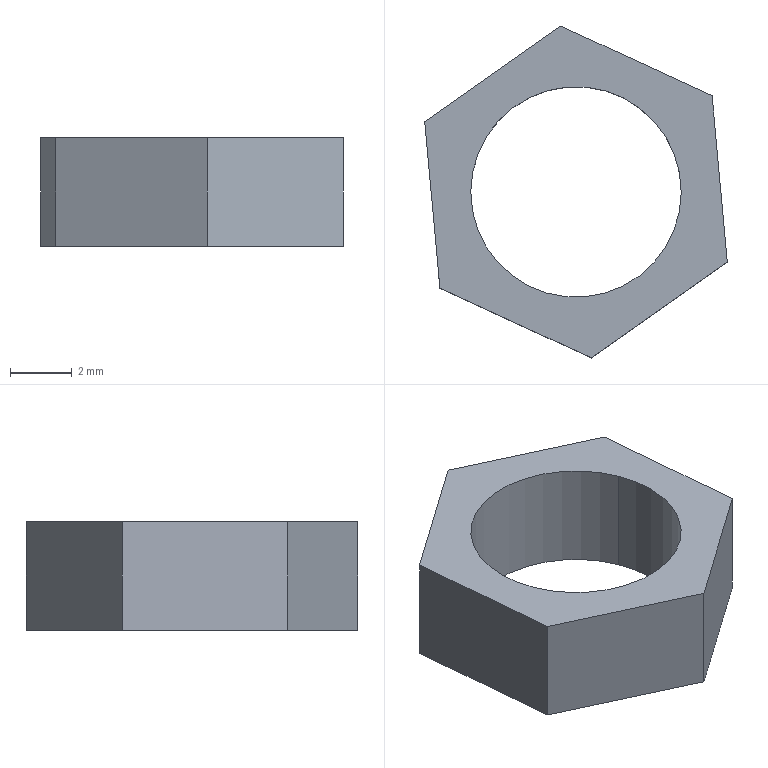Component | SolidWorks | ThinNut-1 | 1 solid | 10 faces | box 9.77 x 10.72 x 3.5 mm | volume 136 mm3 | plane 8 | cylinder 2 | commonest cylinder face diameters 6.8 x2
STEP:
#1=COLOUR_RGB('',0.7922,0.8196,0.9333);
#2=FILL_AREA_STYLE_COLOUR('',#1);
#3=FILL_AREA_STYLE('',(#2));
#4=SURFACE_STYLE_FILL_AREA(#3);
#5=SURFACE_SIDE_STYLE('',(#4));
#6=SURFACE_STYLE_USAGE(.BOTH.,#5);
#7=PRESENTATION_STYLE_ASSIGNMENT((#6));
#8=CARTESIAN_POINT('',(-4.037,-1.074,7.106));
#9=VERTEX_POINT('',#8);
#10=CARTESIAN_POINT('',(-4.287,-1.169,7.106));
#11=VERTEX_POINT('',#10);
#12=CARTESIAN_POINT('',(-4.162,-1.121,7.106));
#13=DIRECTION('',(-0.,0.,-1.));
#14=DIRECTION('',(-0.9336,-0.3582,0.));
#15=AXIS2_PLACEMENT_3D('',#12,#13,#14);
#16=CIRCLE('',#15,0.1339);
#17=EDGE_CURVE('',#9,#11,#16,.T.);
#18=ORIENTED_EDGE('',*,*,#17,.T.);
#19=CARTESIAN_POINT('',(-4.287,-1.169,7.244));
#20=VERTEX_POINT('',#19);
#21=CARTESIAN_POINT('',(-4.287,-1.169,7.106));
#22=DIRECTION('',(0.,-0.,1.));
#23=VECTOR('',#22,39.37);
#24=LINE('',#21,#23);
#25=EDGE_CURVE('',#11,#20,#24,.T.);
#26=ORIENTED_EDGE('',*,*,#25,.T.);
#27=CARTESIAN_POINT('',(-4.037,-1.074,7.244));
#28=VERTEX_POINT('',#27);
#29=CARTESIAN_POINT('',(-4.162,-1.121,7.244));
#30=DIRECTION('',(-0.,0.,-1.));
#31=DIRECTION('',(-0.9336,-0.3582,0.));
#32=AXIS2_PLACEMENT_3D('',#29,#30,#31);
#33=CIRCLE('',#32,0.1339);
#34=EDGE_CURVE('',#28,#20,#33,.T.);
#35=ORIENTED_EDGE('',*,*,#34,.F.);
#36=CARTESIAN_POINT('',(-4.037,-1.074,7.106));
#37=DIRECTION('',(0.,-0.,1.));
#38=VECTOR('',#37,39.37);
#39=LINE('',#36,#38);
#40=EDGE_CURVE('',#9,#28,#39,.T.);
#41=ORIENTED_EDGE('',*,*,#40,.F.);
#42=EDGE_LOOP('',(#18,#26,#35,#41));
#43=FACE_OUTER_BOUND('',#42,.T.);
#44=CARTESIAN_POINT('',(-4.162,-1.121,7.106));
#45=DIRECTION('',(0.,-0.,1.));
#46=DIRECTION('',(0.9336,0.3582,0.));
#47=AXIS2_PLACEMENT_3D('',#44,#45,#46);
#48=CYLINDRICAL_SURFACE('',#47,0.1339);
#49=ADVANCED_FACE('',(#43),#48,.F.);
#50=CARTESIAN_POINT('',(-4.335,-1.244,7.106));
#51=VERTEX_POINT('',#50);
#52=CARTESIAN_POINT('',(-4.355,-1.033,7.106));
#53=VERTEX_POINT('',#52);
#54=CARTESIAN_POINT('',(-4.335,-1.244,7.106));
#55=DIRECTION('',(-0.09039,0.9959,0.));
#56=VECTOR('',#55,39.37);
#57=LINE('',#54,#56);
#58=EDGE_CURVE('',#51,#53,#57,.T.);
#59=ORIENTED_EDGE('',*,*,#58,.T.);
#60=CARTESIAN_POINT('',(-4.181,-0.9104,7.106));
#61=VERTEX_POINT('',#60);
#62=CARTESIAN_POINT('',(-4.355,-1.033,7.106));
#63=DIRECTION('',(0.8173,0.5762,-0.));
#64=VECTOR('',#63,39.37);
#65=LINE('',#62,#64);
#66=EDGE_CURVE('',#53,#61,#65,.T.);
#67=ORIENTED_EDGE('',*,*,#66,.T.);
#68=CARTESIAN_POINT('',(-3.989,-0.9993,7.106));
#69=VERTEX_POINT('',#68);
#70=CARTESIAN_POINT('',(-4.181,-0.9104,7.106));
#71=DIRECTION('',(0.9077,-0.4197,-0.));
#72=VECTOR('',#71,39.37);
#73=LINE('',#70,#72);
#74=EDGE_CURVE('',#61,#69,#73,.T.);
#75=ORIENTED_EDGE('',*,*,#74,.T.);
#76=CARTESIAN_POINT('',(-3.97,-1.21,7.106));
#77=VERTEX_POINT('',#76);
#78=CARTESIAN_POINT('',(-3.989,-0.9993,7.106));
#79=DIRECTION('',(0.09039,-0.9959,-0.));
#80=VECTOR('',#79,39.37);
#81=LINE('',#78,#80);
#82=EDGE_CURVE('',#69,#77,#81,.T.);
#83=ORIENTED_EDGE('',*,*,#82,.T.);
#84=CARTESIAN_POINT('',(-4.143,-1.333,7.106));
#85=VERTEX_POINT('',#84);
#86=CARTESIAN_POINT('',(-3.97,-1.21,7.106));
#87=DIRECTION('',(-0.8173,-0.5762,0.));
#88=VECTOR('',#87,39.37);
#89=LINE('',#86,#88);
#90=EDGE_CURVE('',#77,#85,#89,.T.);
#91=ORIENTED_EDGE('',*,*,#90,.T.);
#92=CARTESIAN_POINT('',(-4.143,-1.333,7.106));
#93=DIRECTION('',(-0.9077,0.4197,0.));
#94=VECTOR('',#93,39.37);
#95=LINE('',#92,#94);
#96=EDGE_CURVE('',#85,#51,#95,.T.);
#97=ORIENTED_EDGE('',*,*,#96,.T.);
#98=EDGE_LOOP('',(#59,#67,#75,#83,#91,#97));
#99=FACE_OUTER_BOUND('',#98,.T.);
#100=ORIENTED_EDGE('',*,*,#17,.F.);
#101=CARTESIAN_POINT('',(-4.162,-1.121,7.106));
#102=DIRECTION('',(-0.,0.,-1.));
#103=DIRECTION('',(-0.9336,-0.3582,0.));
#104=AXIS2_PLACEMENT_3D('',#101,#102,#103);
#105=CIRCLE('',#104,0.1339);
#106=EDGE_CURVE('',#11,#9,#105,.T.);
#107=ORIENTED_EDGE('',*,*,#106,.F.);
#108=EDGE_LOOP('',(#100,#107));
#109=FACE_BOUND('',#108,.T.);
#110=CARTESIAN_POINT('',(-0.678,1.417,7.106));
#111=DIRECTION('',(-0.,0.,-1.));
#112=DIRECTION('',(-0.9336,-0.3582,0.));
#113=AXIS2_PLACEMENT_3D('',#110,#111,#112);
#114=PLANE('',#113);
#115=ADVANCED_FACE('',(#99,#109),#114,.T.);
#116=CARTESIAN_POINT('',(-4.335,-1.244,7.244));
#117=VERTEX_POINT('',#116);
#118=CARTESIAN_POINT('',(-4.355,-1.033,7.244));
#119=VERTEX_POINT('',#118);
#120=CARTESIAN_POINT('',(-4.335,-1.244,7.244));
#121=DIRECTION('',(-0.09039,0.9959,0.));
#122=VECTOR('',#121,39.37);
#123=LINE('',#120,#122);
#124=EDGE_CURVE('',#117,#119,#123,.T.);
#125=ORIENTED_EDGE('',*,*,#124,.F.);
#126=CARTESIAN_POINT('',(-4.143,-1.333,7.244));
#127=VERTEX_POINT('',#126);
#128=CARTESIAN_POINT('',(-4.143,-1.333,7.244));
#129=DIRECTION('',(-0.9077,0.4197,0.));
#130=VECTOR('',#129,39.37);
#131=LINE('',#128,#130);
#132=EDGE_CURVE('',#127,#117,#131,.T.);
#133=ORIENTED_EDGE('',*,*,#132,.F.);
#134=CARTESIAN_POINT('',(-3.97,-1.21,7.244));
#135=VERTEX_POINT('',#134);
#136=CARTESIAN_POINT('',(-3.97,-1.21,7.244));
#137=DIRECTION('',(-0.8173,-0.5762,0.));
#138=VECTOR('',#137,39.37);
#139=LINE('',#136,#138);
#140=EDGE_CURVE('',#135,#127,#139,.T.);
#141=ORIENTED_EDGE('',*,*,#140,.F.);
#142=CARTESIAN_POINT('',(-3.989,-0.9993,7.244));
#143=VERTEX_POINT('',#142);
#144=CARTESIAN_POINT('',(-3.989,-0.9993,7.244));
#145=DIRECTION('',(0.09039,-0.9959,-0.));
#146=VECTOR('',#145,39.37);
#147=LINE('',#144,#146);
#148=EDGE_CURVE('',#143,#135,#147,.T.);
#149=ORIENTED_EDGE('',*,*,#148,.F.);
#150=CARTESIAN_POINT('',(-4.181,-0.9104,7.244));
#151=VERTEX_POINT('',#150);
#152=CARTESIAN_POINT('',(-4.181,-0.9104,7.244));
#153=DIRECTION('',(0.9077,-0.4197,-0.));
#154=VECTOR('',#153,39.37);
#155=LINE('',#152,#154);
#156=EDGE_CURVE('',#151,#143,#155,.T.);
#157=ORIENTED_EDGE('',*,*,#156,.F.);
#158=CARTESIAN_POINT('',(-4.355,-1.033,7.244));
#159=DIRECTION('',(0.8173,0.5762,-0.));
#160=VECTOR('',#159,39.37);
#161=LINE('',#158,#160);
#162=EDGE_CURVE('',#119,#151,#161,.T.);
#163=ORIENTED_EDGE('',*,*,#162,.F.);
#164=EDGE_LOOP('',(#125,#133,#141,#149,#157,#163));
#165=FACE_OUTER_BOUND('',#164,.T.);
#166=ORIENTED_EDGE('',*,*,#34,.T.);
#167=CARTESIAN_POINT('',(-4.162,-1.121,7.244));
#168=DIRECTION('',(-0.,0.,-1.));
#169=DIRECTION('',(-0.9336,-0.3582,0.));
#170=AXIS2_PLACEMENT_3D('',#167,#168,#169);
#171=CIRCLE('',#170,0.1339);
#172=EDGE_CURVE('',#20,#28,#171,.T.);
#173=ORIENTED_EDGE('',*,*,#172,.T.);
#174=EDGE_LOOP('',(#166,#173));
#175=FACE_BOUND('',#174,.T.);
#176=CARTESIAN_POINT('',(-0.678,1.417,7.244));
#177=DIRECTION('',(-0.,0.,-1.));
#178=DIRECTION('',(-0.9336,-0.3582,0.));
#179=AXIS2_PLACEMENT_3D('',#176,#177,#178);
#180=PLANE('',#179);
#181=ADVANCED_FACE('',(#165,#175),#180,.F.);
#182=ORIENTED_EDGE('',*,*,#124,.T.);
#183=CARTESIAN_POINT('',(-4.355,-1.033,7.106));
#184=DIRECTION('',(0.,-0.,1.));
#185=VECTOR('',#184,39.37);
#186=LINE('',#183,#185);
#187=EDGE_CURVE('',#53,#119,#186,.T.);
#188=ORIENTED_EDGE('',*,*,#187,.F.);
#189=ORIENTED_EDGE('',*,*,#58,.F.);
#190=CARTESIAN_POINT('',(-4.335,-1.244,7.106));
#191=DIRECTION('',(0.,-0.,1.));
#192=VECTOR('',#191,39.37);
#193=LINE('',#190,#192);
#194=EDGE_CURVE('',#51,#117,#193,.T.);
#195=ORIENTED_EDGE('',*,*,#194,.T.);
#196=EDGE_LOOP('',(#182,#188,#189,#195));
#197=FACE_OUTER_BOUND('',#196,.T.);
#198=CARTESIAN_POINT('',(-4.335,-1.244,7.106));
#199=DIRECTION('',(0.9959,0.09039,-0.));
#200=DIRECTION('',(0.09039,-0.9959,-0.));
#201=AXIS2_PLACEMENT_3D('',#198,#199,#200);
#202=PLANE('',#201);
#203=ADVANCED_FACE('',(#197),#202,.F.);
#204=ORIENTED_EDGE('',*,*,#162,.T.);
#205=CARTESIAN_POINT('',(-4.181,-0.9104,7.106));
#206=DIRECTION('',(0.,-0.,1.));
#207=VECTOR('',#206,39.37);
#208=LINE('',#205,#207);
#209=EDGE_CURVE('',#61,#151,#208,.T.);
#210=ORIENTED_EDGE('',*,*,#209,.F.);
#211=ORIENTED_EDGE('',*,*,#66,.F.);
#212=ORIENTED_EDGE('',*,*,#187,.T.);
#213=EDGE_LOOP('',(#204,#210,#211,#212));
#214=FACE_OUTER_BOUND('',#213,.T.);
#215=CARTESIAN_POINT('',(-4.355,-1.033,7.106));
#216=DIRECTION('',(0.5762,-0.8173,-0.));
#217=DIRECTION('',(-0.8173,-0.5762,0.));
#218=AXIS2_PLACEMENT_3D('',#215,#216,#217);
#219=PLANE('',#218);
#220=ADVANCED_FACE('',(#214),#219,.F.);
#221=ORIENTED_EDGE('',*,*,#156,.T.);
#222=CARTESIAN_POINT('',(-3.989,-0.9993,7.106));
#223=DIRECTION('',(0.,-0.,1.));
#224=VECTOR('',#223,39.37);
#225=LINE('',#222,#224);
#226=EDGE_CURVE('',#69,#143,#225,.T.);
#227=ORIENTED_EDGE('',*,*,#226,.F.);
#228=ORIENTED_EDGE('',*,*,#74,.F.);
#229=ORIENTED_EDGE('',*,*,#209,.T.);
#230=EDGE_LOOP('',(#221,#227,#228,#229));
#231=FACE_OUTER_BOUND('',#230,.T.);
#232=CARTESIAN_POINT('',(-4.181,-0.9104,7.106));
#233=DIRECTION('',(-0.4197,-0.9077,-0.));
#234=DIRECTION('',(-0.9077,0.4197,0.));
#235=AXIS2_PLACEMENT_3D('',#232,#233,#234);
#236=PLANE('',#235);
#237=ADVANCED_FACE('',(#231),#236,.F.);
#238=ORIENTED_EDGE('',*,*,#148,.T.);
#239=CARTESIAN_POINT('',(-3.97,-1.21,7.106));
#240=DIRECTION('',(0.,-0.,1.));
#241=VECTOR('',#240,39.37);
#242=LINE('',#239,#241);
#243=EDGE_CURVE('',#77,#135,#242,.T.);
#244=ORIENTED_EDGE('',*,*,#243,.F.);
#245=ORIENTED_EDGE('',*,*,#82,.F.);
#246=ORIENTED_EDGE('',*,*,#226,.T.);
#247=EDGE_LOOP('',(#238,#244,#245,#246));
#248=FACE_OUTER_BOUND('',#247,.T.);
#249=CARTESIAN_POINT('',(-3.989,-0.9993,7.106));
#250=DIRECTION('',(-0.9959,-0.09039,0.));
#251=DIRECTION('',(-0.09039,0.9959,0.));
#252=AXIS2_PLACEMENT_3D('',#249,#250,#251);
#253=PLANE('',#252);
#254=ADVANCED_FACE('',(#248),#253,.F.);
#255=ORIENTED_EDGE('',*,*,#140,.T.);
#256=CARTESIAN_POINT('',(-4.143,-1.333,7.106));
#257=DIRECTION('',(0.,-0.,1.));
#258=VECTOR('',#257,39.37);
#259=LINE('',#256,#258);
#260=EDGE_CURVE('',#85,#127,#259,.T.);
#261=ORIENTED_EDGE('',*,*,#260,.F.);
#262=ORIENTED_EDGE('',*,*,#90,.F.);
#263=ORIENTED_EDGE('',*,*,#243,.T.);
#264=EDGE_LOOP('',(#255,#261,#262,#263));
#265=FACE_OUTER_BOUND('',#264,.T.);
#266=CARTESIAN_POINT('',(-3.97,-1.21,7.106));
#267=DIRECTION('',(-0.5762,0.8173,0.));
#268=DIRECTION('',(0.8173,0.5762,-0.));
#269=AXIS2_PLACEMENT_3D('',#266,#267,#268);
#270=PLANE('',#269);
#271=ADVANCED_FACE('',(#265),#270,.F.);
#272=ORIENTED_EDGE('',*,*,#132,.T.);
#273=ORIENTED_EDGE('',*,*,#194,.F.);
#274=ORIENTED_EDGE('',*,*,#96,.F.);
#275=ORIENTED_EDGE('',*,*,#260,.T.);
#276=EDGE_LOOP('',(#272,#273,#274,#275));
#277=FACE_OUTER_BOUND('',#276,.T.);
#278=CARTESIAN_POINT('',(-4.143,-1.333,7.106));
#279=DIRECTION('',(0.4197,0.9077,0.));
#280=DIRECTION('',(0.9077,-0.4197,-0.));
#281=AXIS2_PLACEMENT_3D('',#278,#279,#280);
#282=PLANE('',#281);
#283=ADVANCED_FACE('',(#277),#282,.F.);
#284=ORIENTED_EDGE('',*,*,#25,.F.);
#285=ORIENTED_EDGE('',*,*,#106,.T.);
#286=ORIENTED_EDGE('',*,*,#40,.T.);
#287=ORIENTED_EDGE('',*,*,#172,.F.);
#288=EDGE_LOOP('',(#284,#285,#286,#287));
#289=FACE_OUTER_BOUND('',#288,.T.);
#290=CARTESIAN_POINT('',(-4.162,-1.121,7.106));
#291=DIRECTION('',(0.,-0.,1.));
#292=DIRECTION('',(0.9336,0.3582,0.));
#293=AXIS2_PLACEMENT_3D('',#290,#291,#292);
#294=CYLINDRICAL_SURFACE('',#293,0.1339);
#295=ADVANCED_FACE('',(#289),#294,.F.);
#296=CLOSED_SHELL('',(#49,#115,#181,#203,#220,#237,#254,#271,#283,#295));
#297=MANIFOLD_SOLID_BREP('',#296);
#298=STYLED_ITEM('',(#7),#297);
#299=(LENGTH_UNIT()NAMED_UNIT(*)SI_UNIT($,.METRE.));
#300=LENGTH_MEASURE_WITH_UNIT(LENGTH_MEASURE(0.0254),#299);
#301=DIMENSIONAL_EXPONENTS(1.,0.,0.,0.,0.,0.,0.);
#302=(CONVERSION_BASED_UNIT('',#300)LENGTH_UNIT()NAMED_UNIT(#301));
#303=UNCERTAINTY_MEASURE_WITH_UNIT(LENGTH_MEASURE(0.00001),#302,'','');
#304=(NAMED_UNIT(*)PLANE_ANGLE_UNIT()SI_UNIT($,.RADIAN.));
#305=(NAMED_UNIT(*)SI_UNIT($,.STERADIAN.)SOLID_ANGLE_UNIT());
#306=(GEOMETRIC_REPRESENTATION_CONTEXT(3)GLOBAL_UNCERTAINTY_ASSIGNED_CONTEXT((#303))GLOBAL_UNIT_ASSIGNED_CONTEXT((#302,#304,#305))REPRESENTATION_CONTEXT('',''));
#307=MECHANICAL_DESIGN_GEOMETRIC_PRESENTATION_REPRESENTATION('',(#298),#306);
#308=PRESENTATION_LAYER_ASSIGNMENT('','',(#298));
#309=CARTESIAN_POINT('',(0.,0.,0.));
#310=DIRECTION('',(0.,0.,1.));
#311=DIRECTION('',(1.,0.,0.));
#312=AXIS2_PLACEMENT_3D('',#309,#310,#311);
#313=(LENGTH_UNIT()NAMED_UNIT(*)SI_UNIT($,.METRE.));
#314=LENGTH_MEASURE_WITH_UNIT(LENGTH_MEASURE(0.0254),#313);
#315=DIMENSIONAL_EXPONENTS(1.,0.,0.,0.,0.,0.,0.);
#316=(CONVERSION_BASED_UNIT('',#314)LENGTH_UNIT()NAMED_UNIT(#315));
#317=UNCERTAINTY_MEASURE_WITH_UNIT(LENGTH_MEASURE(0.00001),#316,'','');
#318=(NAMED_UNIT(*)PLANE_ANGLE_UNIT()SI_UNIT($,.RADIAN.));
#319=(NAMED_UNIT(*)SI_UNIT($,.STERADIAN.)SOLID_ANGLE_UNIT());
#320=(GEOMETRIC_REPRESENTATION_CONTEXT(3)GLOBAL_UNCERTAINTY_ASSIGNED_CONTEXT((#317))GLOBAL_UNIT_ASSIGNED_CONTEXT((#316,#318,#319))REPRESENTATION_CONTEXT('',''));
#321=ADVANCED_BREP_SHAPE_REPRESENTATION('',(#297,#312),#320);